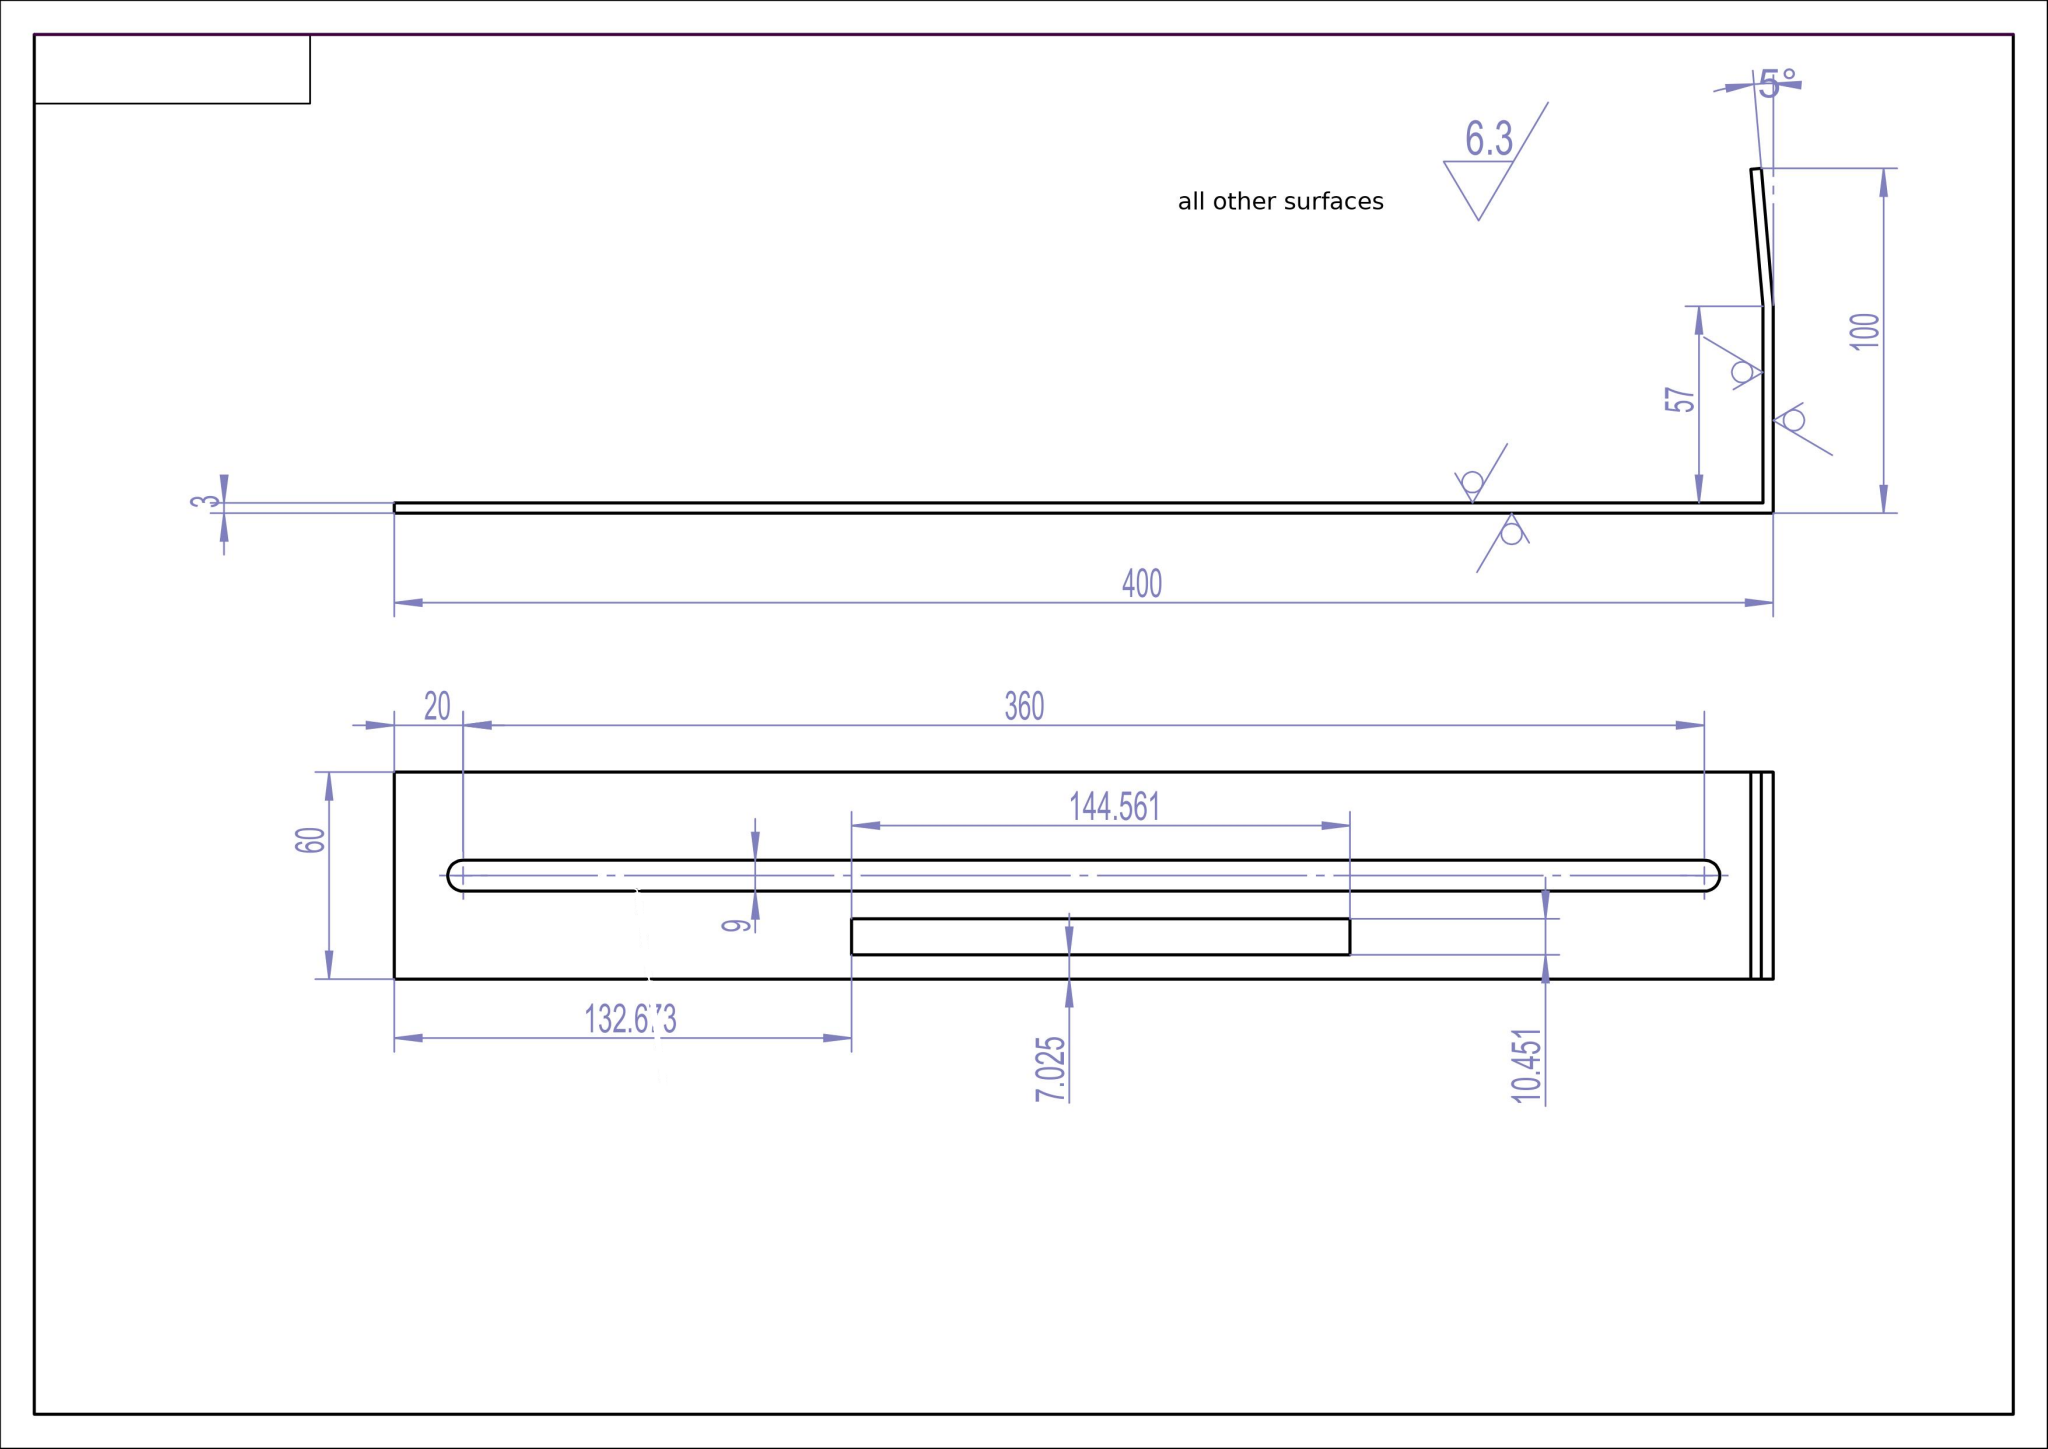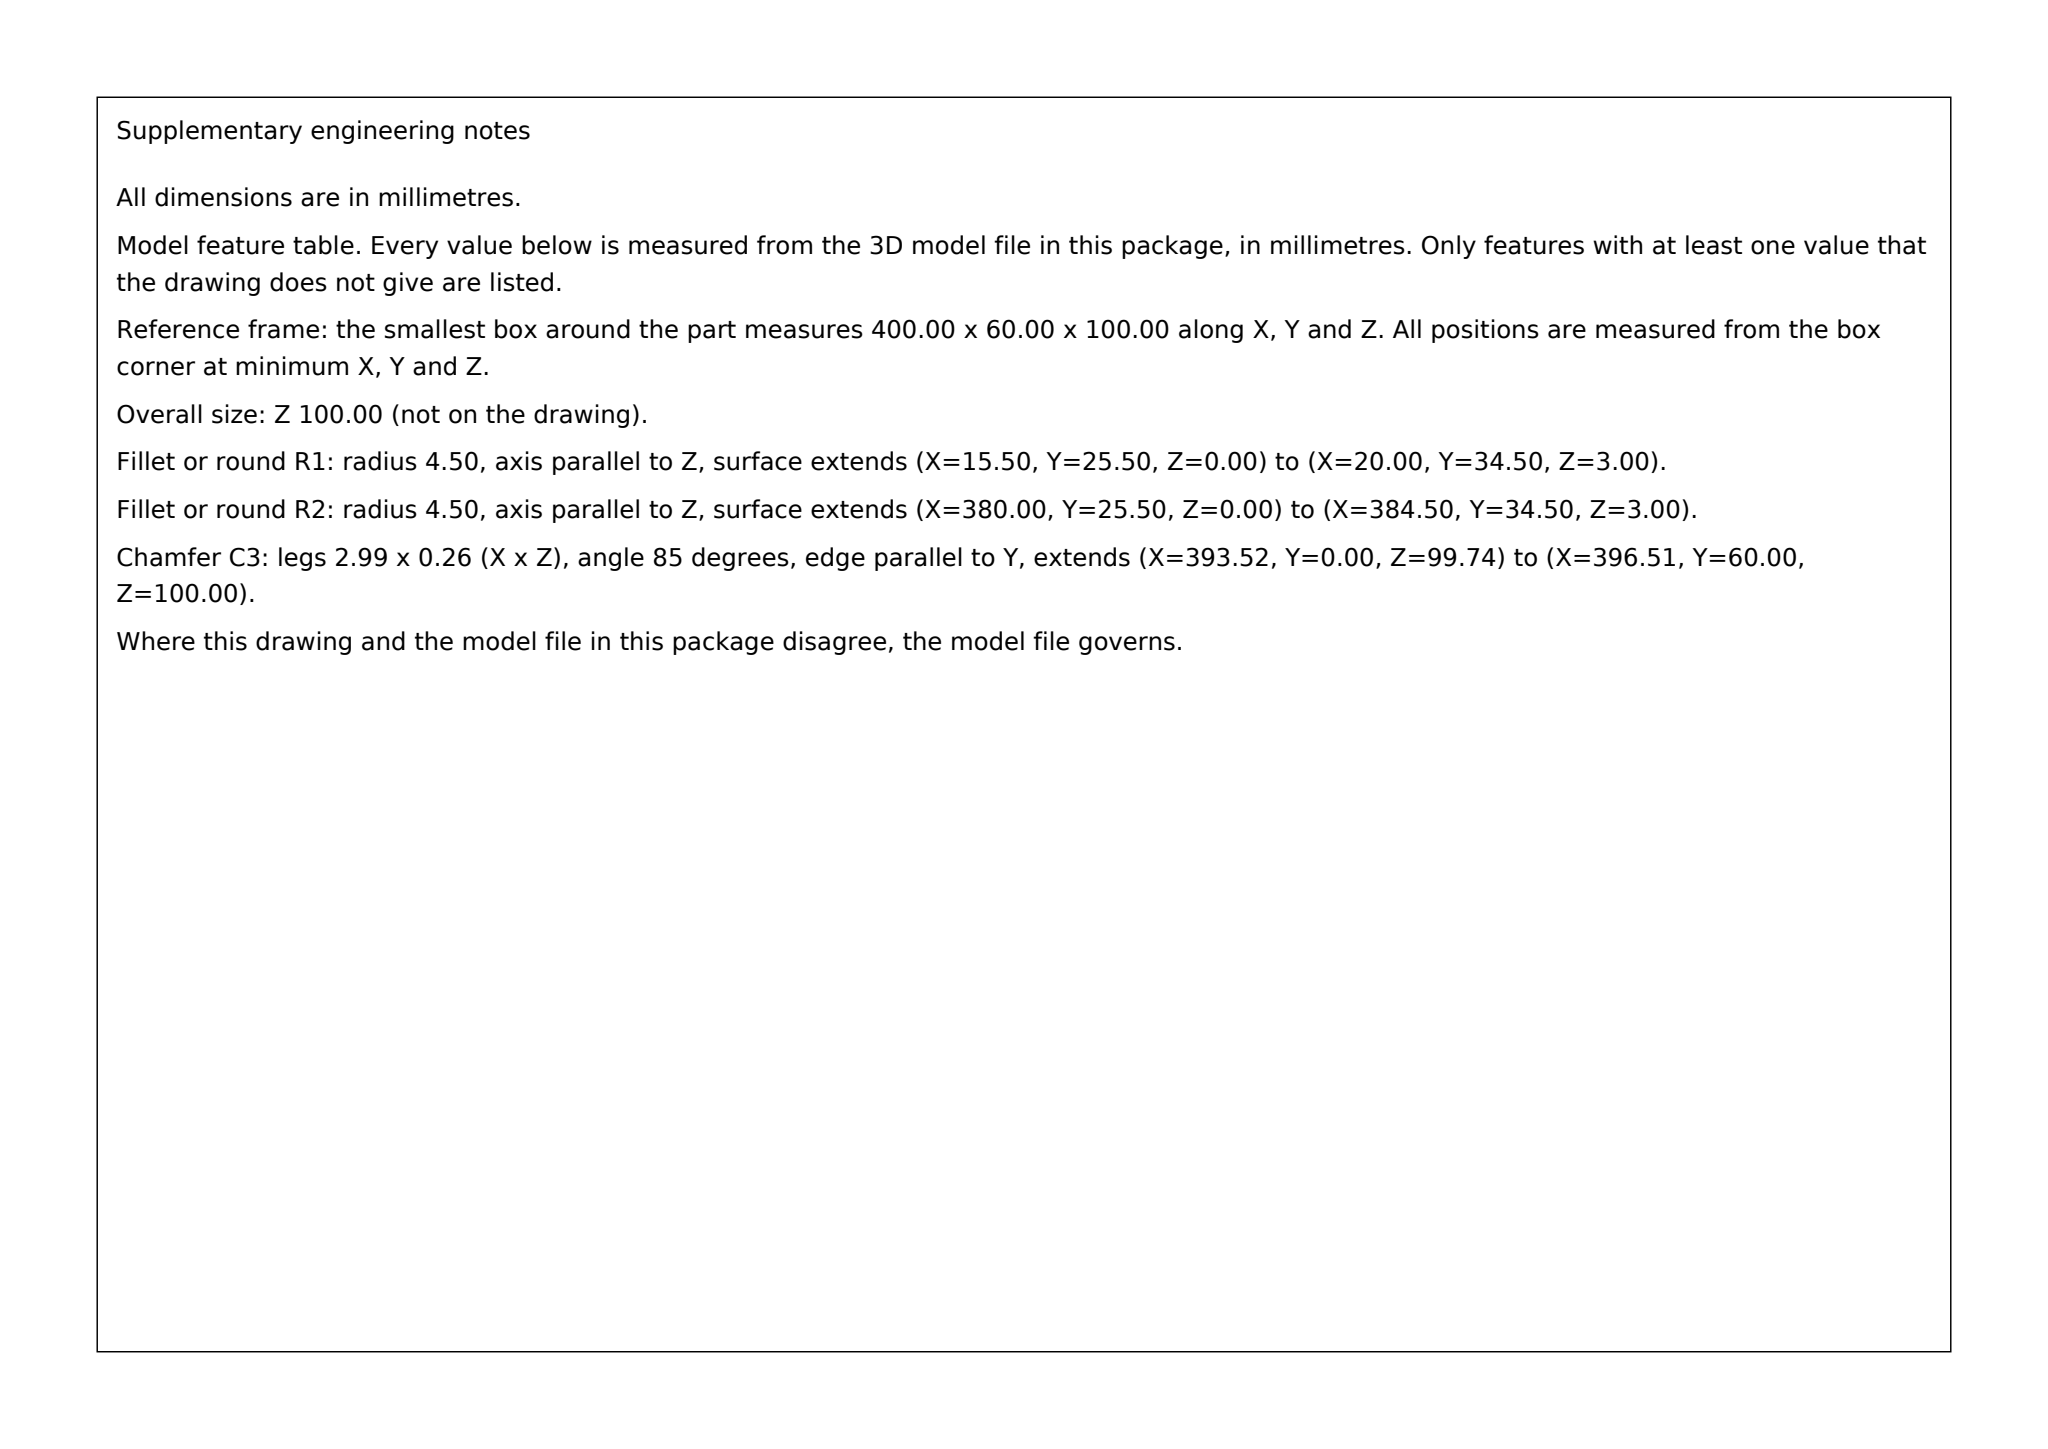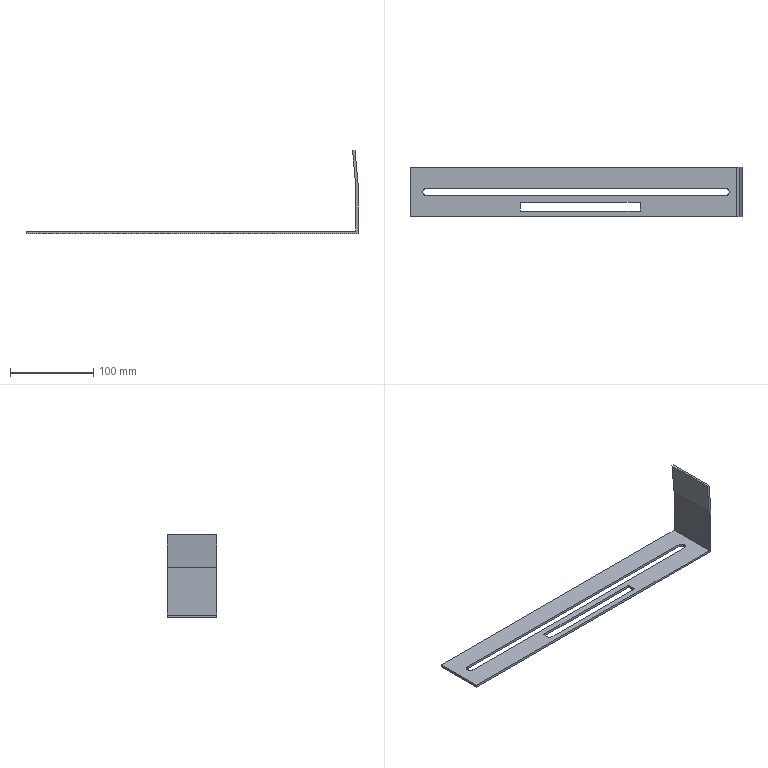Part | SolidWorks | mm | 1 solid | 19 faces | box 400 x 60 x 100 mm | volume 75020 mm3 | plane 16 | cylinder 3 | commonest cylinder face diameters 9 x3
build123d program:
from build123d import *

# Parameters (mm, degrees)
SKETCH1_W           = 400
SKETCH1_H           = 60
BOSS_EXTRUDE1_DEPTH = 3
CUT_EXTRUDE1_DEPTH  = 3
BOSS_EXTRUDE2_DEPTH = 60
SKETCH4_W           = 144.561
SKETCH4_H           = 10.451
CUT_EXTRUDE2_DEPTH  = 60


with BuildPart() as part:
    # Sketch1 → Boss-Extrude1 (new body)
    with BuildSketch(Plane.XY):
        with Locations((112.77, -4.656)):
            Rectangle(SKETCH1_W, SKETCH1_H)
    extrude(amount=BOSS_EXTRUDE1_DEPTH)

    # Sketch2 → Cut-Extrude1 (cut)
    with BuildSketch(Plane.XY.offset(3)):
        with BuildLine():
            Line((-67.23, -0.1562), (292.77, -0.1562))
            ThreePointArc((292.77, -0.1562), (297.27, -4.656), (292.77, -9.156))
            Line((292.77, -9.156), (-67.23, -9.156))
            ThreePointArc((-67.23, -9.156), (-71.73, -4.656), (-67.23, -0.1562))
        make_face()
    extrude(amount=-CUT_EXTRUDE1_DEPTH, mode=Mode.SUBTRACT)

    # Sketch3 → Boss-Extrude2 (add)
    with BuildSketch(Plane.XZ.offset(34.656)):
        Polygon((312.77, 3), (312.77, 60.131), (309.282, 100), (306.293, 99.739), (309.77, 60), (309.77, 3), align=None)
    extrude(amount=-BOSS_EXTRUDE2_DEPTH)

    # Sketch4 → Cut-Extrude2 (cut)
    with BuildSketch(Plane.XY.offset(3)):
        with Locations((117.724, -22.406)):
            Rectangle(SKETCH4_W, SKETCH4_H)
    extrude(amount=-CUT_EXTRUDE2_DEPTH, mode=Mode.SUBTRACT)


solid = part.part
STEP:
#1=CARTESIAN_POINT('',(297.27,-4.656,0.));
#2=VERTEX_POINT('',#1);
#3=CARTESIAN_POINT('',(292.77,-0.1562,0.));
#4=VERTEX_POINT('',#3);
#5=CARTESIAN_POINT('',(292.77,-4.656,0.));
#6=DIRECTION('',(0.,0.,1.));
#7=DIRECTION('',(1.,0.,0.));
#8=AXIS2_PLACEMENT_3D('',#5,#6,#7);
#9=CIRCLE('',#8,4.5);
#10=EDGE_CURVE('',#2,#4,#9,.T.);
#11=ORIENTED_EDGE('',*,*,#10,.F.);
#12=CARTESIAN_POINT('',(297.27,-4.656,3.));
#13=VERTEX_POINT('',#12);
#14=CARTESIAN_POINT('',(297.27,-4.656,0.));
#15=DIRECTION('',(0.,0.,1.));
#16=VECTOR('',#15,1000.);
#17=LINE('',#14,#16);
#18=EDGE_CURVE('',#2,#13,#17,.T.);
#19=ORIENTED_EDGE('',*,*,#18,.T.);
#20=CARTESIAN_POINT('',(292.77,-0.1562,3.));
#21=VERTEX_POINT('',#20);
#22=CARTESIAN_POINT('',(292.77,-4.656,3.));
#23=DIRECTION('',(0.,0.,1.));
#24=DIRECTION('',(1.,0.,0.));
#25=AXIS2_PLACEMENT_3D('',#22,#23,#24);
#26=CIRCLE('',#25,4.5);
#27=EDGE_CURVE('',#13,#21,#26,.T.);
#28=ORIENTED_EDGE('',*,*,#27,.T.);
#29=CARTESIAN_POINT('',(292.77,-0.1562,0.));
#30=DIRECTION('',(0.,0.,1.));
#31=VECTOR('',#30,1000.);
#32=LINE('',#29,#31);
#33=EDGE_CURVE('',#4,#21,#32,.T.);
#34=ORIENTED_EDGE('',*,*,#33,.F.);
#35=EDGE_LOOP('',(#11,#19,#28,#34));
#36=FACE_OUTER_BOUND('',#35,.T.);
#37=CARTESIAN_POINT('',(292.77,-4.656,0.));
#38=DIRECTION('',(0.,0.,1.));
#39=DIRECTION('',(1.,0.,0.));
#40=AXIS2_PLACEMENT_3D('',#37,#38,#39);
#41=CYLINDRICAL_SURFACE('',#40,4.5);
#42=ADVANCED_FACE('',(#36),#41,.F.);
#43=CARTESIAN_POINT('',(-87.23,25.344,0.));
#44=VERTEX_POINT('',#43);
#45=CARTESIAN_POINT('',(-87.23,-34.656,0.));
#46=VERTEX_POINT('',#45);
#47=CARTESIAN_POINT('',(-87.23,25.344,0.));
#48=DIRECTION('',(0.,-1.,0.));
#49=VECTOR('',#48,1000.);
#50=LINE('',#47,#49);
#51=EDGE_CURVE('',#44,#46,#50,.T.);
#52=ORIENTED_EDGE('',*,*,#51,.T.);
#53=CARTESIAN_POINT('',(-87.23,-34.656,3.));
#54=VERTEX_POINT('',#53);
#55=CARTESIAN_POINT('',(-87.23,-34.656,3.));
#56=DIRECTION('',(0.,0.,-1.));
#57=VECTOR('',#56,1000.);
#58=LINE('',#55,#57);
#59=EDGE_CURVE('',#54,#46,#58,.T.);
#60=ORIENTED_EDGE('',*,*,#59,.F.);
#61=CARTESIAN_POINT('',(-87.23,25.344,3.));
#62=VERTEX_POINT('',#61);
#63=CARTESIAN_POINT('',(-87.23,25.344,3.));
#64=DIRECTION('',(0.,-1.,0.));
#65=VECTOR('',#64,1000.);
#66=LINE('',#63,#65);
#67=EDGE_CURVE('',#62,#54,#66,.T.);
#68=ORIENTED_EDGE('',*,*,#67,.F.);
#69=CARTESIAN_POINT('',(-87.23,25.344,3.));
#70=DIRECTION('',(0.,0.,-1.));
#71=VECTOR('',#70,1000.);
#72=LINE('',#69,#71);
#73=EDGE_CURVE('',#62,#44,#72,.T.);
#74=ORIENTED_EDGE('',*,*,#73,.T.);
#75=EDGE_LOOP('',(#52,#60,#68,#74));
#76=FACE_OUTER_BOUND('',#75,.T.);
#77=CARTESIAN_POINT('',(-87.23,25.344,3.));
#78=DIRECTION('',(1.,0.,0.));
#79=DIRECTION('',(-0.,1.,0.));
#80=AXIS2_PLACEMENT_3D('',#77,#78,#79);
#81=PLANE('',#80);
#82=ADVANCED_FACE('',(#76),#81,.F.);
#83=CARTESIAN_POINT('',(312.77,-34.656,0.));
#84=VERTEX_POINT('',#83);
#85=CARTESIAN_POINT('',(-87.23,-34.656,0.));
#86=DIRECTION('',(1.,0.,0.));
#87=VECTOR('',#86,1000.);
#88=LINE('',#85,#87);
#89=EDGE_CURVE('',#46,#84,#88,.T.);
#90=ORIENTED_EDGE('',*,*,#89,.T.);
#91=CARTESIAN_POINT('',(312.77,-34.656,60.131));
#92=VERTEX_POINT('',#91);
#93=CARTESIAN_POINT('',(312.77,-34.656,3.));
#94=DIRECTION('',(0.,0.,-1.));
#95=VECTOR('',#94,1000.);
#96=LINE('',#93,#95);
#97=EDGE_CURVE('',#92,#84,#96,.T.);
#98=ORIENTED_EDGE('',*,*,#97,.F.);
#99=CARTESIAN_POINT('',(309.282,-34.656,100.));
#100=VERTEX_POINT('',#99);
#101=CARTESIAN_POINT('',(309.282,-34.656,100.));
#102=DIRECTION('',(-0.08716,0.,0.9962));
#103=VECTOR('',#102,1000.);
#104=LINE('',#101,#103);
#105=EDGE_CURVE('',#92,#100,#104,.T.);
#106=ORIENTED_EDGE('',*,*,#105,.T.);
#107=CARTESIAN_POINT('',(306.293,-34.656,99.739));
#108=VERTEX_POINT('',#107);
#109=CARTESIAN_POINT('',(306.293,-34.656,99.739));
#110=DIRECTION('',(-0.9962,0.,-0.08716));
#111=VECTOR('',#110,1000.);
#112=LINE('',#109,#111);
#113=EDGE_CURVE('',#100,#108,#112,.T.);
#114=ORIENTED_EDGE('',*,*,#113,.T.);
#115=CARTESIAN_POINT('',(309.77,-34.656,60.));
#116=VERTEX_POINT('',#115);
#117=CARTESIAN_POINT('',(309.77,-34.656,60.));
#118=DIRECTION('',(0.08716,0.,-0.9962));
#119=VECTOR('',#118,1000.);
#120=LINE('',#117,#119);
#121=EDGE_CURVE('',#108,#116,#120,.T.);
#122=ORIENTED_EDGE('',*,*,#121,.T.);
#123=CARTESIAN_POINT('',(309.77,-34.656,3.));
#124=VERTEX_POINT('',#123);
#125=CARTESIAN_POINT('',(309.77,-34.656,3.));
#126=DIRECTION('',(0.,0.,-1.));
#127=VECTOR('',#126,1000.);
#128=LINE('',#125,#127);
#129=EDGE_CURVE('',#116,#124,#128,.T.);
#130=ORIENTED_EDGE('',*,*,#129,.T.);
#131=CARTESIAN_POINT('',(-87.23,-34.656,3.));
#132=DIRECTION('',(1.,0.,0.));
#133=VECTOR('',#132,1000.);
#134=LINE('',#131,#133);
#135=EDGE_CURVE('',#54,#124,#134,.T.);
#136=ORIENTED_EDGE('',*,*,#135,.F.);
#137=ORIENTED_EDGE('',*,*,#59,.T.);
#138=EDGE_LOOP('',(#90,#98,#106,#114,#122,#130,#136,#137));
#139=FACE_OUTER_BOUND('',#138,.T.);
#140=CARTESIAN_POINT('',(-87.23,-34.656,3.));
#141=DIRECTION('',(0.,1.,0.));
#142=DIRECTION('',(0.,0.,1.));
#143=AXIS2_PLACEMENT_3D('',#140,#141,#142);
#144=PLANE('',#143);
#145=ADVANCED_FACE('',(#139),#144,.F.);
#146=CARTESIAN_POINT('',(312.77,25.344,0.));
#147=VERTEX_POINT('',#146);
#148=CARTESIAN_POINT('',(312.77,25.344,0.));
#149=DIRECTION('',(0.,1.,0.));
#150=VECTOR('',#149,1000.);
#151=LINE('',#148,#150);
#152=EDGE_CURVE('',#84,#147,#151,.T.);
#153=ORIENTED_EDGE('',*,*,#152,.T.);
#154=CARTESIAN_POINT('',(312.77,25.344,60.131));
#155=VERTEX_POINT('',#154);
#156=CARTESIAN_POINT('',(312.77,25.344,3.));
#157=DIRECTION('',(0.,0.,-1.));
#158=VECTOR('',#157,1000.);
#159=LINE('',#156,#158);
#160=EDGE_CURVE('',#155,#147,#159,.T.);
#161=ORIENTED_EDGE('',*,*,#160,.F.);
#162=CARTESIAN_POINT('',(312.77,25.344,60.131));
#163=DIRECTION('',(0.,-1.,0.));
#164=VECTOR('',#163,1000.);
#165=LINE('',#162,#164);
#166=EDGE_CURVE('',#155,#92,#165,.T.);
#167=ORIENTED_EDGE('',*,*,#166,.T.);
#168=ORIENTED_EDGE('',*,*,#97,.T.);
#169=EDGE_LOOP('',(#153,#161,#167,#168));
#170=FACE_OUTER_BOUND('',#169,.T.);
#171=CARTESIAN_POINT('',(312.77,25.344,3.));
#172=DIRECTION('',(-1.,0.,0.));
#173=DIRECTION('',(0.,0.,1.));
#174=AXIS2_PLACEMENT_3D('',#171,#172,#173);
#175=PLANE('',#174);
#176=ADVANCED_FACE('',(#170),#175,.F.);
#177=CARTESIAN_POINT('',(-87.23,25.344,0.));
#178=DIRECTION('',(-1.,0.,0.));
#179=VECTOR('',#178,1000.);
#180=LINE('',#177,#179);
#181=EDGE_CURVE('',#147,#44,#180,.T.);
#182=ORIENTED_EDGE('',*,*,#181,.T.);
#183=ORIENTED_EDGE('',*,*,#73,.F.);
#184=CARTESIAN_POINT('',(309.77,25.344,3.));
#185=VERTEX_POINT('',#184);
#186=CARTESIAN_POINT('',(-87.23,25.344,3.));
#187=DIRECTION('',(-1.,0.,0.));
#188=VECTOR('',#187,1000.);
#189=LINE('',#186,#188);
#190=EDGE_CURVE('',#185,#62,#189,.T.);
#191=ORIENTED_EDGE('',*,*,#190,.F.);
#192=CARTESIAN_POINT('',(309.77,25.344,60.));
#193=VERTEX_POINT('',#192);
#194=CARTESIAN_POINT('',(309.77,25.344,3.));
#195=DIRECTION('',(0.,0.,-1.));
#196=VECTOR('',#195,1000.);
#197=LINE('',#194,#196);
#198=EDGE_CURVE('',#193,#185,#197,.T.);
#199=ORIENTED_EDGE('',*,*,#198,.F.);
#200=CARTESIAN_POINT('',(306.293,25.344,99.739));
#201=VERTEX_POINT('',#200);
#202=CARTESIAN_POINT('',(309.77,25.344,60.));
#203=DIRECTION('',(0.08716,0.,-0.9962));
#204=VECTOR('',#203,1000.);
#205=LINE('',#202,#204);
#206=EDGE_CURVE('',#201,#193,#205,.T.);
#207=ORIENTED_EDGE('',*,*,#206,.F.);
#208=CARTESIAN_POINT('',(309.282,25.344,100.));
#209=VERTEX_POINT('',#208);
#210=CARTESIAN_POINT('',(306.293,25.344,99.739));
#211=DIRECTION('',(-0.9962,0.,-0.08716));
#212=VECTOR('',#211,1000.);
#213=LINE('',#210,#212);
#214=EDGE_CURVE('',#209,#201,#213,.T.);
#215=ORIENTED_EDGE('',*,*,#214,.F.);
#216=CARTESIAN_POINT('',(309.282,25.344,100.));
#217=DIRECTION('',(-0.08716,0.,0.9962));
#218=VECTOR('',#217,1000.);
#219=LINE('',#216,#218);
#220=EDGE_CURVE('',#155,#209,#219,.T.);
#221=ORIENTED_EDGE('',*,*,#220,.F.);
#222=ORIENTED_EDGE('',*,*,#160,.T.);
#223=EDGE_LOOP('',(#182,#183,#191,#199,#207,#215,#221,#222));
#224=FACE_OUTER_BOUND('',#223,.T.);
#225=CARTESIAN_POINT('',(-87.23,25.344,3.));
#226=DIRECTION('',(0.,-1.,0.));
#227=DIRECTION('',(0.,0.,-1.));
#228=AXIS2_PLACEMENT_3D('',#225,#226,#227);
#229=PLANE('',#228);
#230=ADVANCED_FACE('',(#224),#229,.F.);
#231=CARTESIAN_POINT('',(45.443,-17.18,3.));
#232=VERTEX_POINT('',#231);
#233=CARTESIAN_POINT('',(45.443,-27.631,3.));
#234=VERTEX_POINT('',#233);
#235=CARTESIAN_POINT('',(45.443,-17.18,3.));
#236=DIRECTION('',(0.,-1.,0.));
#237=VECTOR('',#236,1000.);
#238=LINE('',#235,#237);
#239=EDGE_CURVE('',#232,#234,#238,.T.);
#240=ORIENTED_EDGE('',*,*,#239,.F.);
#241=CARTESIAN_POINT('',(190.004,-17.18,3.));
#242=VERTEX_POINT('',#241);
#243=CARTESIAN_POINT('',(45.443,-17.18,3.));
#244=DIRECTION('',(-1.,0.,0.));
#245=VECTOR('',#244,1000.);
#246=LINE('',#243,#245);
#247=EDGE_CURVE('',#242,#232,#246,.T.);
#248=ORIENTED_EDGE('',*,*,#247,.F.);
#249=CARTESIAN_POINT('',(190.004,-27.631,3.));
#250=VERTEX_POINT('',#249);
#251=CARTESIAN_POINT('',(190.004,-17.18,3.));
#252=DIRECTION('',(0.,1.,0.));
#253=VECTOR('',#252,1000.);
#254=LINE('',#251,#253);
#255=EDGE_CURVE('',#250,#242,#254,.T.);
#256=ORIENTED_EDGE('',*,*,#255,.F.);
#257=CARTESIAN_POINT('',(45.443,-27.631,3.));
#258=DIRECTION('',(1.,0.,0.));
#259=VECTOR('',#258,1000.);
#260=LINE('',#257,#259);
#261=EDGE_CURVE('',#234,#250,#260,.T.);
#262=ORIENTED_EDGE('',*,*,#261,.F.);
#263=EDGE_LOOP('',(#240,#248,#256,#262));
#264=FACE_BOUND('',#263,.T.);
#265=CARTESIAN_POINT('',(309.77,25.344,3.));
#266=DIRECTION('',(0.,-1.,0.));
#267=VECTOR('',#266,1000.);
#268=LINE('',#265,#267);
#269=EDGE_CURVE('',#185,#124,#268,.T.);
#270=ORIENTED_EDGE('',*,*,#269,.F.);
#271=ORIENTED_EDGE('',*,*,#190,.T.);
#272=ORIENTED_EDGE('',*,*,#67,.T.);
#273=ORIENTED_EDGE('',*,*,#135,.T.);
#274=EDGE_LOOP('',(#270,#271,#272,#273));
#275=FACE_OUTER_BOUND('',#274,.T.);
#276=CARTESIAN_POINT('',(-67.23,-0.1562,3.));
#277=VERTEX_POINT('',#276);
#278=CARTESIAN_POINT('',(-67.23,-9.156,3.));
#279=VERTEX_POINT('',#278);
#280=CARTESIAN_POINT('',(-67.23,-4.656,3.));
#281=DIRECTION('',(0.,0.,1.));
#282=DIRECTION('',(1.,0.,0.));
#283=AXIS2_PLACEMENT_3D('',#280,#281,#282);
#284=CIRCLE('',#283,4.5);
#285=EDGE_CURVE('',#277,#279,#284,.T.);
#286=ORIENTED_EDGE('',*,*,#285,.F.);
#287=CARTESIAN_POINT('',(-67.23,-0.1562,3.));
#288=DIRECTION('',(-1.,0.,0.));
#289=VECTOR('',#288,1000.);
#290=LINE('',#287,#289);
#291=EDGE_CURVE('',#21,#277,#290,.T.);
#292=ORIENTED_EDGE('',*,*,#291,.F.);
#293=ORIENTED_EDGE('',*,*,#27,.F.);
#294=CARTESIAN_POINT('',(292.77,-9.156,3.));
#295=VERTEX_POINT('',#294);
#296=CARTESIAN_POINT('',(292.77,-4.656,3.));
#297=DIRECTION('',(0.,0.,1.));
#298=DIRECTION('',(1.,0.,0.));
#299=AXIS2_PLACEMENT_3D('',#296,#297,#298);
#300=CIRCLE('',#299,4.5);
#301=EDGE_CURVE('',#295,#13,#300,.T.);
#302=ORIENTED_EDGE('',*,*,#301,.F.);
#303=CARTESIAN_POINT('',(-67.23,-9.156,3.));
#304=DIRECTION('',(1.,0.,0.));
#305=VECTOR('',#304,1000.);
#306=LINE('',#303,#305);
#307=EDGE_CURVE('',#279,#295,#306,.T.);
#308=ORIENTED_EDGE('',*,*,#307,.F.);
#309=EDGE_LOOP('',(#286,#292,#293,#302,#308));
#310=FACE_BOUND('',#309,.T.);
#311=CARTESIAN_POINT('',(0.,0.,3.));
#312=DIRECTION('',(0.,0.,1.));
#313=DIRECTION('',(1.,0.,0.));
#314=AXIS2_PLACEMENT_3D('',#311,#312,#313);
#315=PLANE('',#314);
#316=ADVANCED_FACE('',(#264,#275,#310),#315,.T.);
#317=CARTESIAN_POINT('',(190.004,-17.18,0.));
#318=VERTEX_POINT('',#317);
#319=CARTESIAN_POINT('',(45.443,-17.18,0.));
#320=VERTEX_POINT('',#319);
#321=CARTESIAN_POINT('',(0.,-17.18,0.));
#322=DIRECTION('',(-1.,0.,0.));
#323=VECTOR('',#322,1000.);
#324=LINE('',#321,#323);
#325=EDGE_CURVE('',#318,#320,#324,.T.);
#326=ORIENTED_EDGE('',*,*,#325,.T.);
#327=CARTESIAN_POINT('',(45.443,-27.631,0.));
#328=VERTEX_POINT('',#327);
#329=CARTESIAN_POINT('',(45.443,0.,0.));
#330=DIRECTION('',(0.,-1.,0.));
#331=VECTOR('',#330,1000.);
#332=LINE('',#329,#331);
#333=EDGE_CURVE('',#320,#328,#332,.T.);
#334=ORIENTED_EDGE('',*,*,#333,.T.);
#335=CARTESIAN_POINT('',(190.004,-27.631,0.));
#336=VERTEX_POINT('',#335);
#337=CARTESIAN_POINT('',(0.,-27.631,0.));
#338=DIRECTION('',(1.,0.,0.));
#339=VECTOR('',#338,1000.);
#340=LINE('',#337,#339);
#341=EDGE_CURVE('',#328,#336,#340,.T.);
#342=ORIENTED_EDGE('',*,*,#341,.T.);
#343=CARTESIAN_POINT('',(190.004,0.,0.));
#344=DIRECTION('',(0.,1.,0.));
#345=VECTOR('',#344,1000.);
#346=LINE('',#343,#345);
#347=EDGE_CURVE('',#336,#318,#346,.T.);
#348=ORIENTED_EDGE('',*,*,#347,.T.);
#349=EDGE_LOOP('',(#326,#334,#342,#348));
#350=FACE_BOUND('',#349,.T.);
#351=CARTESIAN_POINT('',(-67.23,-0.1562,0.));
#352=VERTEX_POINT('',#351);
#353=CARTESIAN_POINT('',(-67.23,-0.1562,0.));
#354=DIRECTION('',(-1.,0.,0.));
#355=VECTOR('',#354,1000.);
#356=LINE('',#353,#355);
#357=EDGE_CURVE('',#4,#352,#356,.T.);
#358=ORIENTED_EDGE('',*,*,#357,.T.);
#359=CARTESIAN_POINT('',(-67.23,-9.156,0.));
#360=VERTEX_POINT('',#359);
#361=CARTESIAN_POINT('',(-67.23,-4.656,0.));
#362=DIRECTION('',(0.,0.,1.));
#363=DIRECTION('',(1.,0.,0.));
#364=AXIS2_PLACEMENT_3D('',#361,#362,#363);
#365=CIRCLE('',#364,4.5);
#366=EDGE_CURVE('',#352,#360,#365,.T.);
#367=ORIENTED_EDGE('',*,*,#366,.T.);
#368=CARTESIAN_POINT('',(292.77,-9.156,0.));
#369=VERTEX_POINT('',#368);
#370=CARTESIAN_POINT('',(-67.23,-9.156,0.));
#371=DIRECTION('',(1.,0.,0.));
#372=VECTOR('',#371,1000.);
#373=LINE('',#370,#372);
#374=EDGE_CURVE('',#360,#369,#373,.T.);
#375=ORIENTED_EDGE('',*,*,#374,.T.);
#376=CARTESIAN_POINT('',(292.77,-4.656,0.));
#377=DIRECTION('',(0.,0.,1.));
#378=DIRECTION('',(1.,0.,0.));
#379=AXIS2_PLACEMENT_3D('',#376,#377,#378);
#380=CIRCLE('',#379,4.5);
#381=EDGE_CURVE('',#369,#2,#380,.T.);
#382=ORIENTED_EDGE('',*,*,#381,.T.);
#383=ORIENTED_EDGE('',*,*,#10,.T.);
#384=EDGE_LOOP('',(#358,#367,#375,#382,#383));
#385=FACE_BOUND('',#384,.T.);
#386=ORIENTED_EDGE('',*,*,#51,.F.);
#387=ORIENTED_EDGE('',*,*,#181,.F.);
#388=ORIENTED_EDGE('',*,*,#152,.F.);
#389=ORIENTED_EDGE('',*,*,#89,.F.);
#390=EDGE_LOOP('',(#386,#387,#388,#389));
#391=FACE_OUTER_BOUND('',#390,.T.);
#392=CARTESIAN_POINT('',(0.,0.,0.));
#393=DIRECTION('',(0.,0.,1.));
#394=DIRECTION('',(1.,0.,0.));
#395=AXIS2_PLACEMENT_3D('',#392,#393,#394);
#396=PLANE('',#395);
#397=ADVANCED_FACE('',(#350,#385,#391),#396,.F.);
#398=ORIENTED_EDGE('',*,*,#285,.T.);
#399=CARTESIAN_POINT('',(-67.23,-9.156,0.));
#400=DIRECTION('',(0.,0.,1.));
#401=VECTOR('',#400,1000.);
#402=LINE('',#399,#401);
#403=EDGE_CURVE('',#360,#279,#402,.T.);
#404=ORIENTED_EDGE('',*,*,#403,.F.);
#405=ORIENTED_EDGE('',*,*,#366,.F.);
#406=CARTESIAN_POINT('',(-67.23,-0.1562,0.));
#407=DIRECTION('',(0.,0.,1.));
#408=VECTOR('',#407,1000.);
#409=LINE('',#406,#408);
#410=EDGE_CURVE('',#352,#277,#409,.T.);
#411=ORIENTED_EDGE('',*,*,#410,.T.);
#412=EDGE_LOOP('',(#398,#404,#405,#411));
#413=FACE_OUTER_BOUND('',#412,.T.);
#414=CARTESIAN_POINT('',(-67.23,-4.656,0.));
#415=DIRECTION('',(0.,0.,1.));
#416=DIRECTION('',(1.,0.,0.));
#417=AXIS2_PLACEMENT_3D('',#414,#415,#416);
#418=CYLINDRICAL_SURFACE('',#417,4.5);
#419=ADVANCED_FACE('',(#413),#418,.F.);
#420=ORIENTED_EDGE('',*,*,#291,.T.);
#421=ORIENTED_EDGE('',*,*,#410,.F.);
#422=ORIENTED_EDGE('',*,*,#357,.F.);
#423=ORIENTED_EDGE('',*,*,#33,.T.);
#424=EDGE_LOOP('',(#420,#421,#422,#423));
#425=FACE_OUTER_BOUND('',#424,.T.);
#426=CARTESIAN_POINT('',(-67.23,-0.1562,0.));
#427=DIRECTION('',(0.,1.,0.));
#428=DIRECTION('',(0.,0.,1.));
#429=AXIS2_PLACEMENT_3D('',#426,#427,#428);
#430=PLANE('',#429);
#431=ADVANCED_FACE('',(#425),#430,.F.);
#432=ORIENTED_EDGE('',*,*,#18,.F.);
#433=ORIENTED_EDGE('',*,*,#381,.F.);
#434=CARTESIAN_POINT('',(292.77,-9.156,0.));
#435=DIRECTION('',(0.,0.,1.));
#436=VECTOR('',#435,1000.);
#437=LINE('',#434,#436);
#438=EDGE_CURVE('',#369,#295,#437,.T.);
#439=ORIENTED_EDGE('',*,*,#438,.T.);
#440=ORIENTED_EDGE('',*,*,#301,.T.);
#441=EDGE_LOOP('',(#432,#433,#439,#440));
#442=FACE_OUTER_BOUND('',#441,.T.);
#443=CARTESIAN_POINT('',(292.77,-4.656,0.));
#444=DIRECTION('',(0.,0.,1.));
#445=DIRECTION('',(1.,0.,0.));
#446=AXIS2_PLACEMENT_3D('',#443,#444,#445);
#447=CYLINDRICAL_SURFACE('',#446,4.5);
#448=ADVANCED_FACE('',(#442),#447,.F.);
#449=ORIENTED_EDGE('',*,*,#307,.T.);
#450=ORIENTED_EDGE('',*,*,#438,.F.);
#451=ORIENTED_EDGE('',*,*,#374,.F.);
#452=ORIENTED_EDGE('',*,*,#403,.T.);
#453=EDGE_LOOP('',(#449,#450,#451,#452));
#454=FACE_OUTER_BOUND('',#453,.T.);
#455=CARTESIAN_POINT('',(-67.23,-9.156,0.));
#456=DIRECTION('',(0.,-1.,0.));
#457=DIRECTION('',(0.,0.,-1.));
#458=AXIS2_PLACEMENT_3D('',#455,#456,#457);
#459=PLANE('',#458);
#460=ADVANCED_FACE('',(#454),#459,.F.);
#461=ORIENTED_EDGE('',*,*,#129,.F.);
#462=CARTESIAN_POINT('',(309.77,25.344,60.));
#463=DIRECTION('',(0.,-1.,0.));
#464=VECTOR('',#463,1000.);
#465=LINE('',#462,#464);
#466=EDGE_CURVE('',#193,#116,#465,.T.);
#467=ORIENTED_EDGE('',*,*,#466,.F.);
#468=ORIENTED_EDGE('',*,*,#198,.T.);
#469=ORIENTED_EDGE('',*,*,#269,.T.);
#470=EDGE_LOOP('',(#461,#467,#468,#469));
#471=FACE_OUTER_BOUND('',#470,.T.);
#472=CARTESIAN_POINT('',(309.77,25.344,3.));
#473=DIRECTION('',(-1.,0.,0.));
#474=DIRECTION('',(0.,0.,1.));
#475=AXIS2_PLACEMENT_3D('',#472,#473,#474);
#476=PLANE('',#475);
#477=ADVANCED_FACE('',(#471),#476,.T.);
#478=ORIENTED_EDGE('',*,*,#121,.F.);
#479=CARTESIAN_POINT('',(306.293,25.344,99.739));
#480=DIRECTION('',(0.,-1.,0.));
#481=VECTOR('',#480,1000.);
#482=LINE('',#479,#481);
#483=EDGE_CURVE('',#201,#108,#482,.T.);
#484=ORIENTED_EDGE('',*,*,#483,.F.);
#485=ORIENTED_EDGE('',*,*,#206,.T.);
#486=ORIENTED_EDGE('',*,*,#466,.T.);
#487=EDGE_LOOP('',(#478,#484,#485,#486));
#488=FACE_OUTER_BOUND('',#487,.T.);
#489=CARTESIAN_POINT('',(309.77,25.344,60.));
#490=DIRECTION('',(-0.9962,0.,-0.08716));
#491=DIRECTION('',(-0.08716,0.,0.9962));
#492=AXIS2_PLACEMENT_3D('',#489,#490,#491);
#493=PLANE('',#492);
#494=ADVANCED_FACE('',(#488),#493,.T.);
#495=ORIENTED_EDGE('',*,*,#113,.F.);
#496=CARTESIAN_POINT('',(309.282,25.344,100.));
#497=DIRECTION('',(0.,-1.,0.));
#498=VECTOR('',#497,1000.);
#499=LINE('',#496,#498);
#500=EDGE_CURVE('',#209,#100,#499,.T.);
#501=ORIENTED_EDGE('',*,*,#500,.F.);
#502=ORIENTED_EDGE('',*,*,#214,.T.);
#503=ORIENTED_EDGE('',*,*,#483,.T.);
#504=EDGE_LOOP('',(#495,#501,#502,#503));
#505=FACE_OUTER_BOUND('',#504,.T.);
#506=CARTESIAN_POINT('',(306.293,25.344,99.739));
#507=DIRECTION('',(-0.08716,0.,0.9962));
#508=DIRECTION('',(0.9962,0.,0.08716));
#509=AXIS2_PLACEMENT_3D('',#506,#507,#508);
#510=PLANE('',#509);
#511=ADVANCED_FACE('',(#505),#510,.T.);
#512=ORIENTED_EDGE('',*,*,#105,.F.);
#513=ORIENTED_EDGE('',*,*,#166,.F.);
#514=ORIENTED_EDGE('',*,*,#220,.T.);
#515=ORIENTED_EDGE('',*,*,#500,.T.);
#516=EDGE_LOOP('',(#512,#513,#514,#515));
#517=FACE_OUTER_BOUND('',#516,.T.);
#518=CARTESIAN_POINT('',(309.282,25.344,100.));
#519=DIRECTION('',(0.9962,0.,0.08716));
#520=DIRECTION('',(0.08716,0.,-0.9962));
#521=AXIS2_PLACEMENT_3D('',#518,#519,#520);
#522=PLANE('',#521);
#523=ADVANCED_FACE('',(#517),#522,.T.);
#524=CARTESIAN_POINT('',(45.443,-17.18,-57.));
#525=DIRECTION('',(0.,0.,1.));
#526=VECTOR('',#525,1000.);
#527=LINE('',#524,#526);
#528=EDGE_CURVE('',#320,#232,#527,.T.);
#529=ORIENTED_EDGE('',*,*,#528,.T.);
#530=ORIENTED_EDGE('',*,*,#239,.T.);
#531=CARTESIAN_POINT('',(45.443,-27.631,-57.));
#532=DIRECTION('',(0.,0.,1.));
#533=VECTOR('',#532,1000.);
#534=LINE('',#531,#533);
#535=EDGE_CURVE('',#328,#234,#534,.T.);
#536=ORIENTED_EDGE('',*,*,#535,.F.);
#537=ORIENTED_EDGE('',*,*,#333,.F.);
#538=EDGE_LOOP('',(#529,#530,#536,#537));
#539=FACE_OUTER_BOUND('',#538,.T.);
#540=CARTESIAN_POINT('',(45.443,-17.18,-57.));
#541=DIRECTION('',(-1.,0.,0.));
#542=DIRECTION('',(0.,0.,1.));
#543=AXIS2_PLACEMENT_3D('',#540,#541,#542);
#544=PLANE('',#543);
#545=ADVANCED_FACE('',(#539),#544,.F.);
#546=CARTESIAN_POINT('',(190.004,-17.18,-57.));
#547=DIRECTION('',(0.,0.,1.));
#548=VECTOR('',#547,1000.);
#549=LINE('',#546,#548);
#550=EDGE_CURVE('',#318,#242,#549,.T.);
#551=ORIENTED_EDGE('',*,*,#550,.T.);
#552=ORIENTED_EDGE('',*,*,#247,.T.);
#553=ORIENTED_EDGE('',*,*,#528,.F.);
#554=ORIENTED_EDGE('',*,*,#325,.F.);
#555=EDGE_LOOP('',(#551,#552,#553,#554));
#556=FACE_OUTER_BOUND('',#555,.T.);
#557=CARTESIAN_POINT('',(45.443,-17.18,-57.));
#558=DIRECTION('',(0.,1.,0.));
#559=DIRECTION('',(0.,0.,1.));
#560=AXIS2_PLACEMENT_3D('',#557,#558,#559);
#561=PLANE('',#560);
#562=ADVANCED_FACE('',(#556),#561,.F.);
#563=CARTESIAN_POINT('',(190.004,-27.631,-57.));
#564=DIRECTION('',(0.,0.,1.));
#565=VECTOR('',#564,1000.);
#566=LINE('',#563,#565);
#567=EDGE_CURVE('',#336,#250,#566,.T.);
#568=ORIENTED_EDGE('',*,*,#567,.T.);
#569=ORIENTED_EDGE('',*,*,#255,.T.);
#570=ORIENTED_EDGE('',*,*,#550,.F.);
#571=ORIENTED_EDGE('',*,*,#347,.F.);
#572=EDGE_LOOP('',(#568,#569,#570,#571));
#573=FACE_OUTER_BOUND('',#572,.T.);
#574=CARTESIAN_POINT('',(190.004,-17.18,-57.));
#575=DIRECTION('',(1.,0.,0.));
#576=DIRECTION('',(0.,0.,-1.));
#577=AXIS2_PLACEMENT_3D('',#574,#575,#576);
#578=PLANE('',#577);
#579=ADVANCED_FACE('',(#573),#578,.F.);
#580=ORIENTED_EDGE('',*,*,#535,.T.);
#581=ORIENTED_EDGE('',*,*,#261,.T.);
#582=ORIENTED_EDGE('',*,*,#567,.F.);
#583=ORIENTED_EDGE('',*,*,#341,.F.);
#584=EDGE_LOOP('',(#580,#581,#582,#583));
#585=FACE_OUTER_BOUND('',#584,.T.);
#586=CARTESIAN_POINT('',(45.443,-27.631,-57.));
#587=DIRECTION('',(0.,-1.,0.));
#588=DIRECTION('',(0.,0.,-1.));
#589=AXIS2_PLACEMENT_3D('',#586,#587,#588);
#590=PLANE('',#589);
#591=ADVANCED_FACE('',(#585),#590,.F.);
#592=CLOSED_SHELL('',(#42,#82,#145,#176,#230,#316,#397,#419,#431,#448,#460,#477,#494,#511,#523,#545,#562,#579,#591));
#593=MANIFOLD_SOLID_BREP('',#592);
#594=CARTESIAN_POINT('',(0.,0.,0.));
#595=DIRECTION('',(0.,0.,1.));
#596=DIRECTION('',(1.,0.,0.));
#597=AXIS2_PLACEMENT_3D('',#594,#595,#596);
#598=(LENGTH_UNIT()NAMED_UNIT(*)SI_UNIT(.MILLI.,.METRE.));
#599=UNCERTAINTY_MEASURE_WITH_UNIT(LENGTH_MEASURE(0.00001),#598,'','');
#600=(NAMED_UNIT(*)PLANE_ANGLE_UNIT()SI_UNIT($,.RADIAN.));
#601=(NAMED_UNIT(*)SI_UNIT($,.STERADIAN.)SOLID_ANGLE_UNIT());
#602=(GEOMETRIC_REPRESENTATION_CONTEXT(3)GLOBAL_UNCERTAINTY_ASSIGNED_CONTEXT((#599))GLOBAL_UNIT_ASSIGNED_CONTEXT((#598,#600,#601))REPRESENTATION_CONTEXT('',''));
#603=ADVANCED_BREP_SHAPE_REPRESENTATION('',(#593,#597),#602);